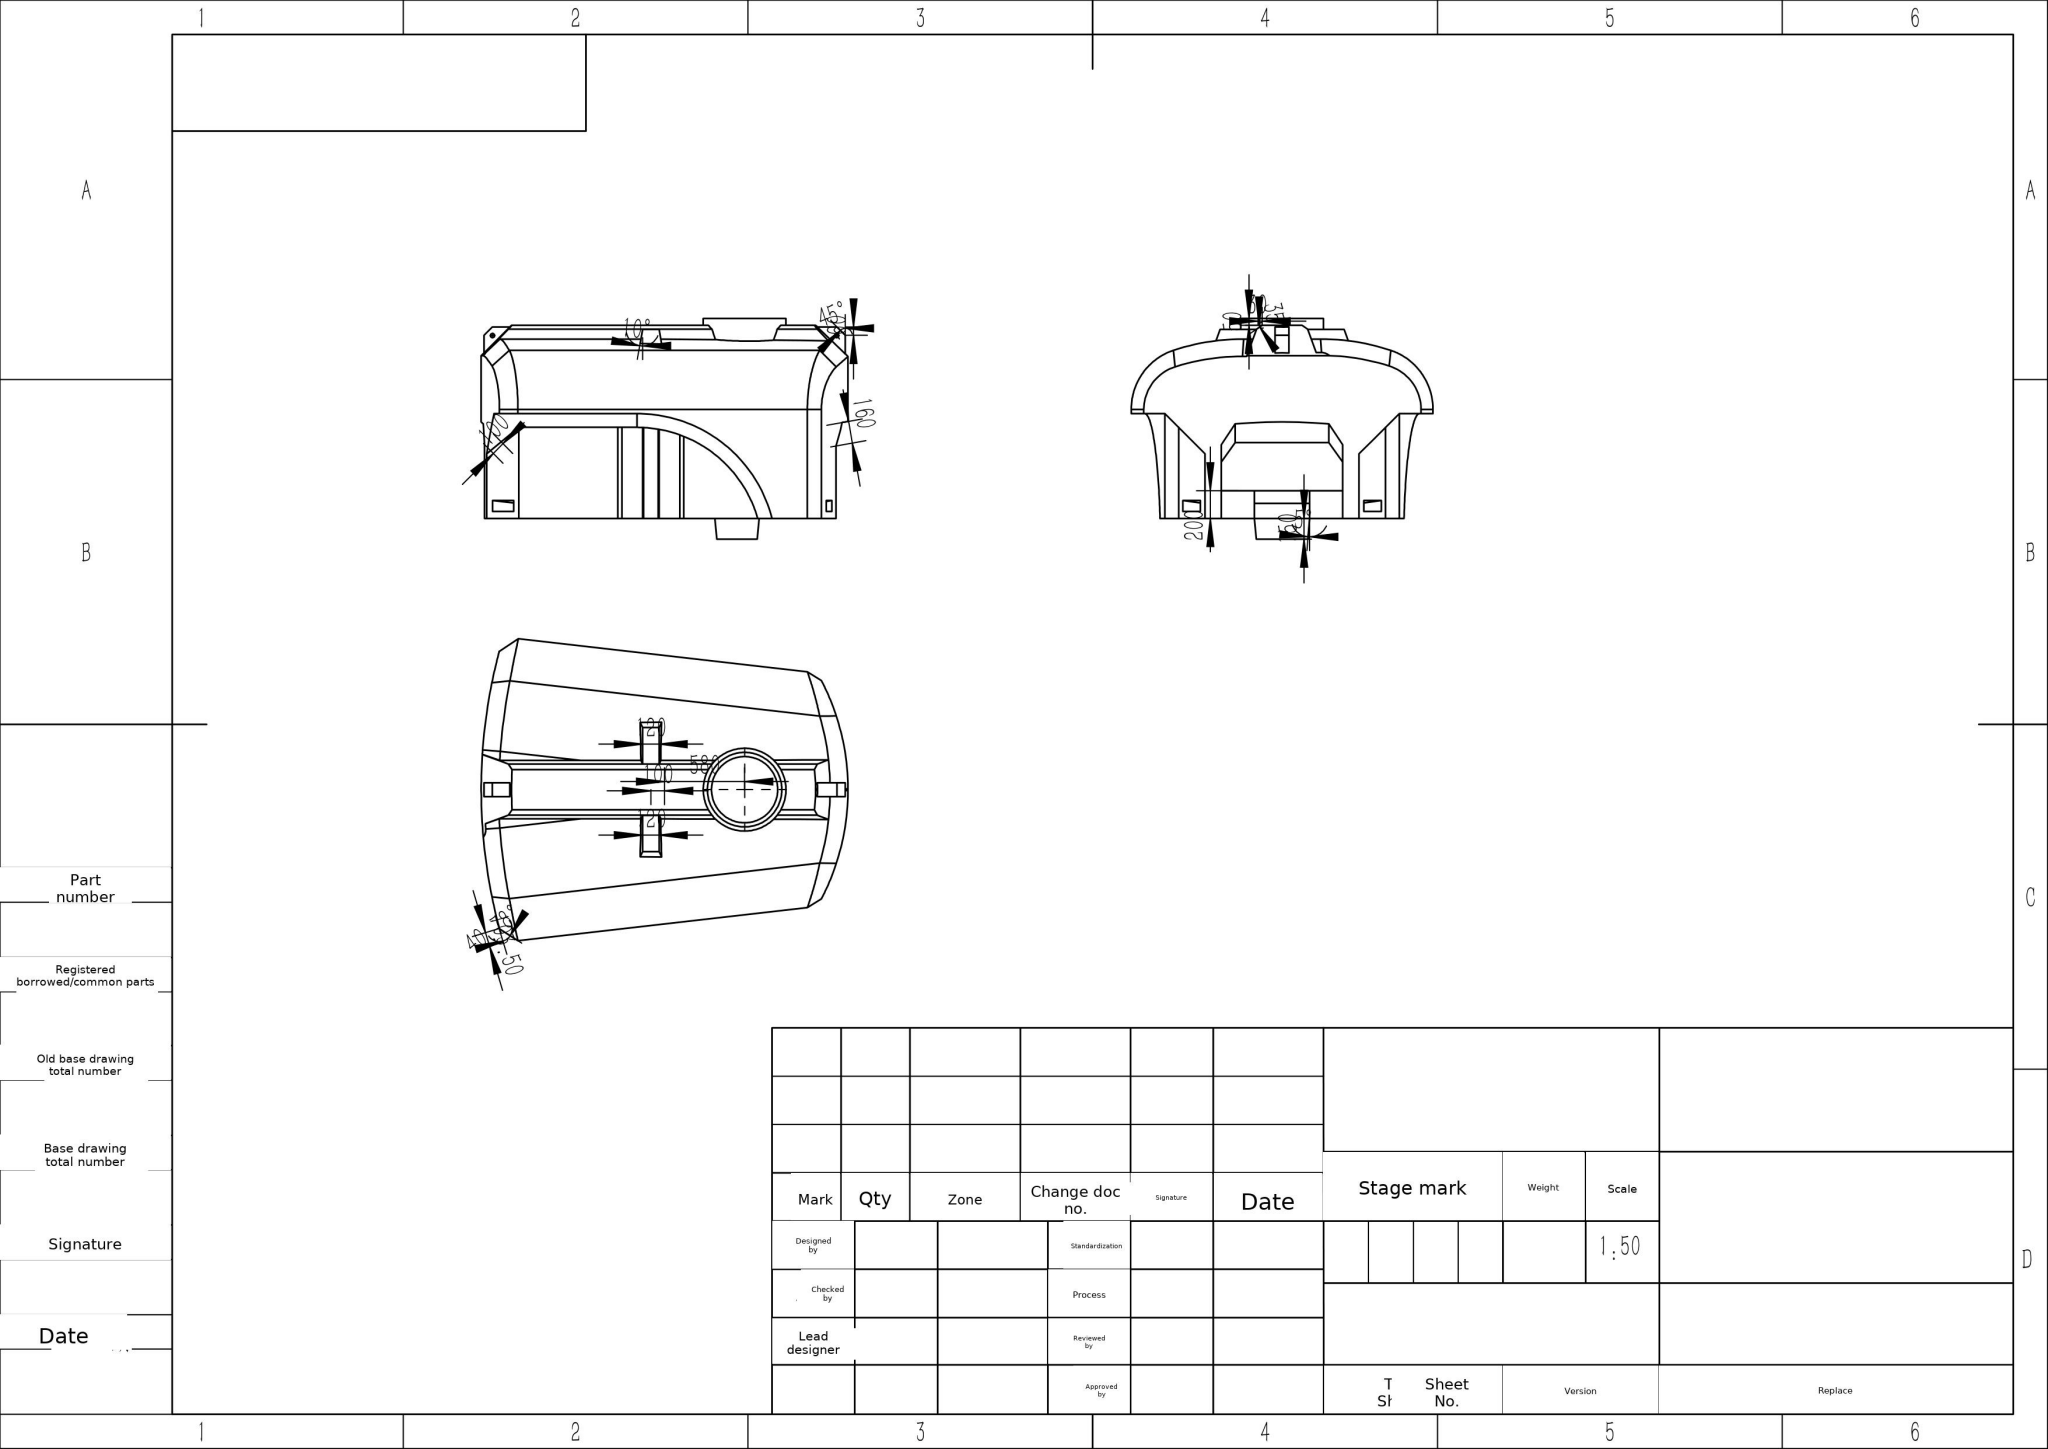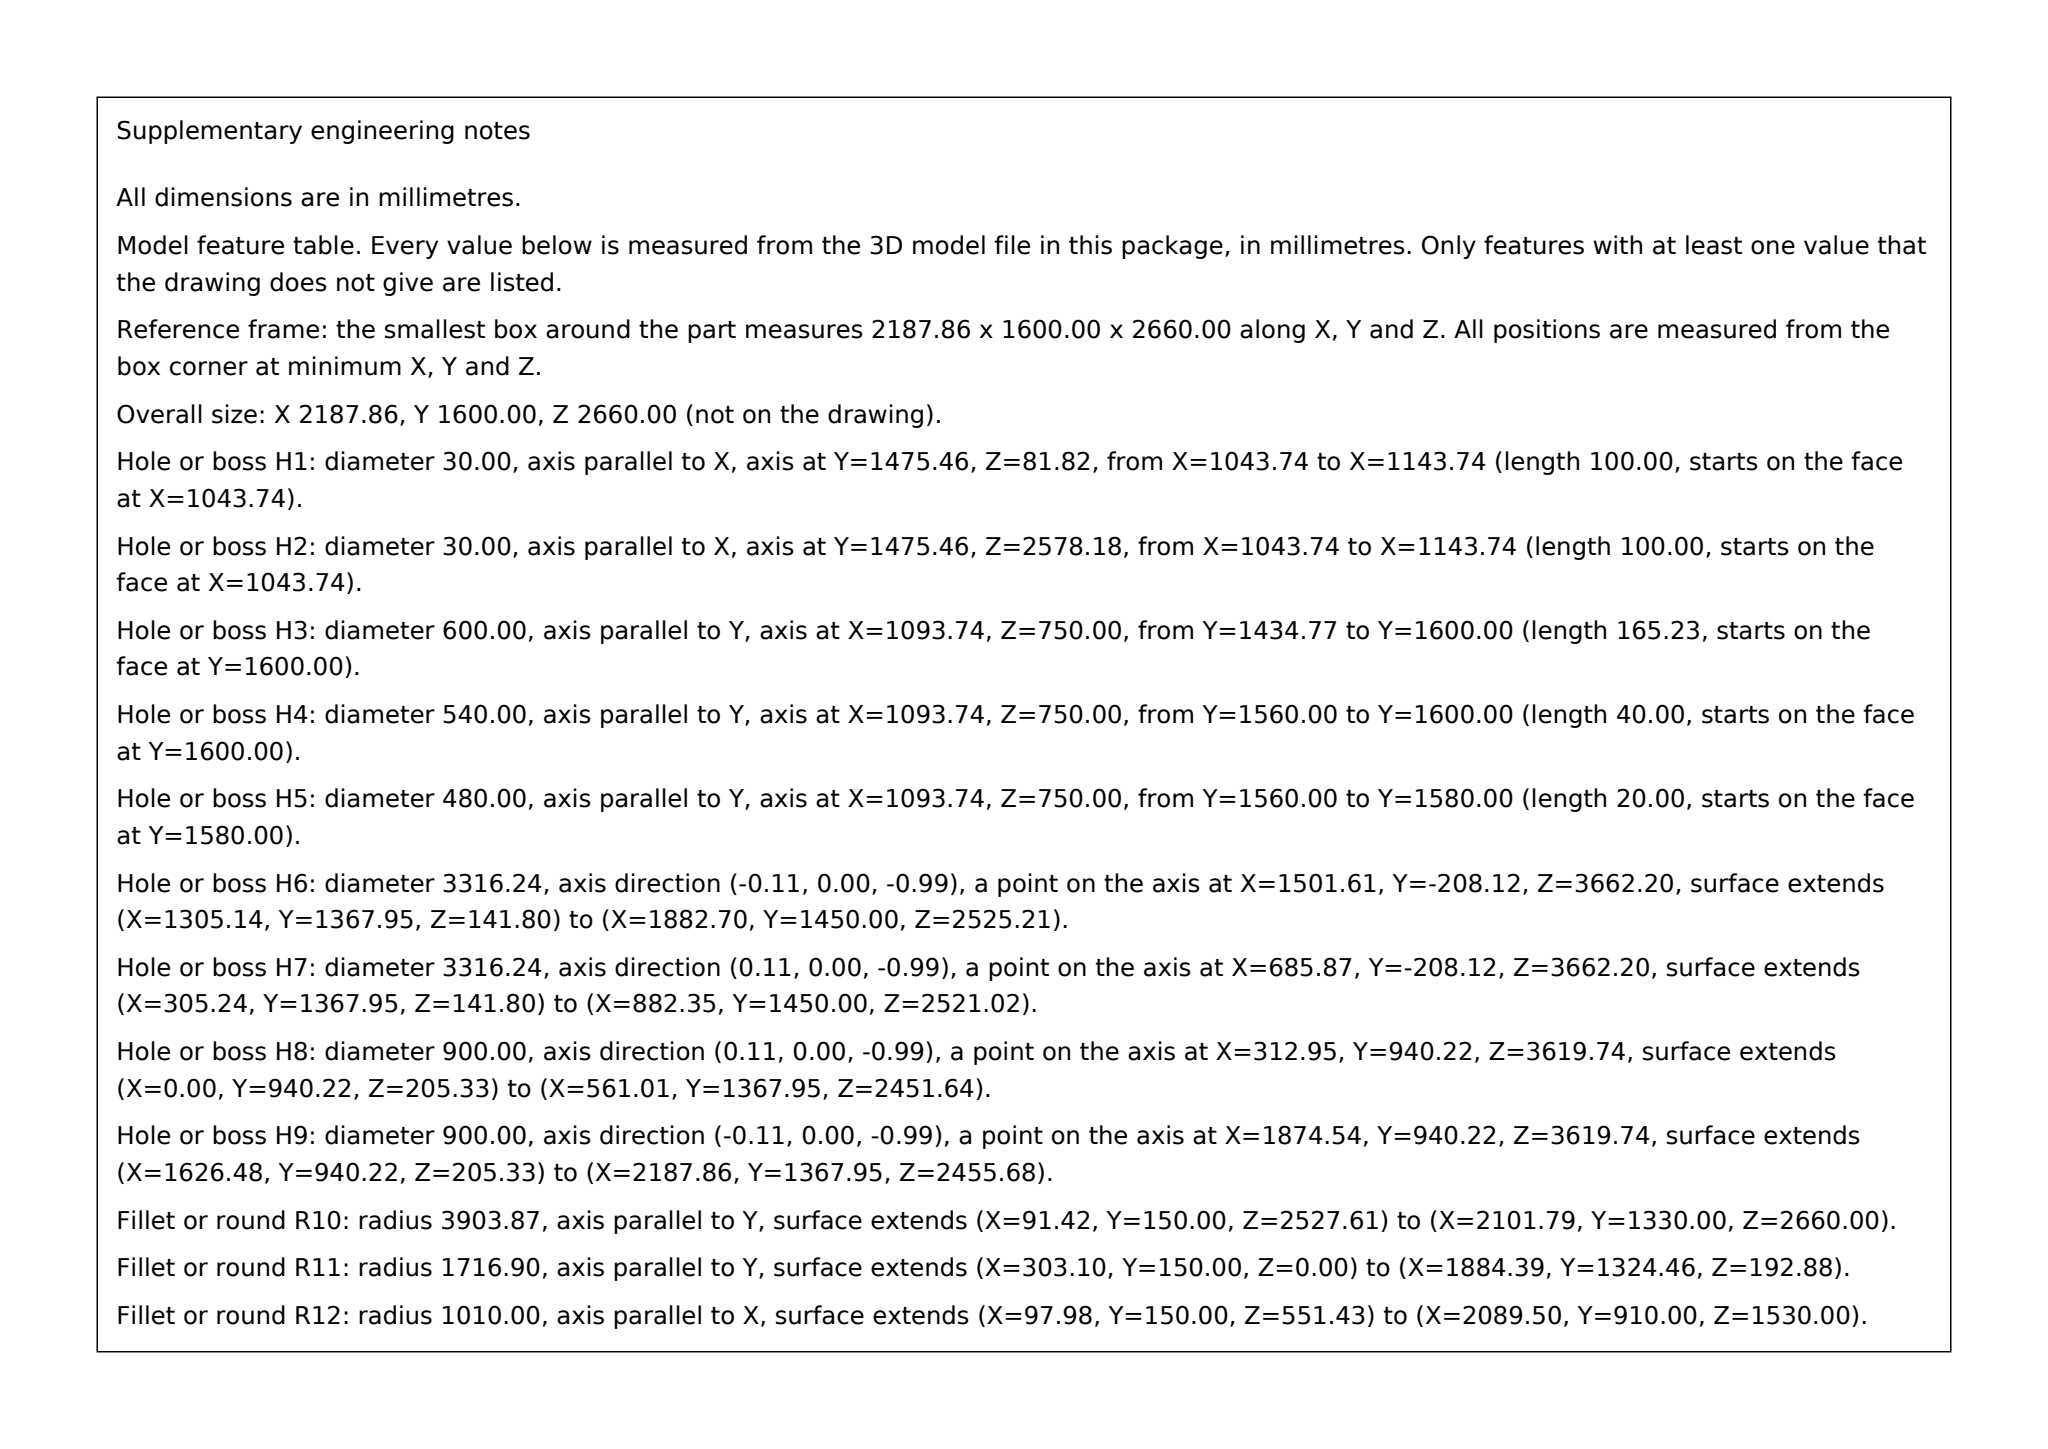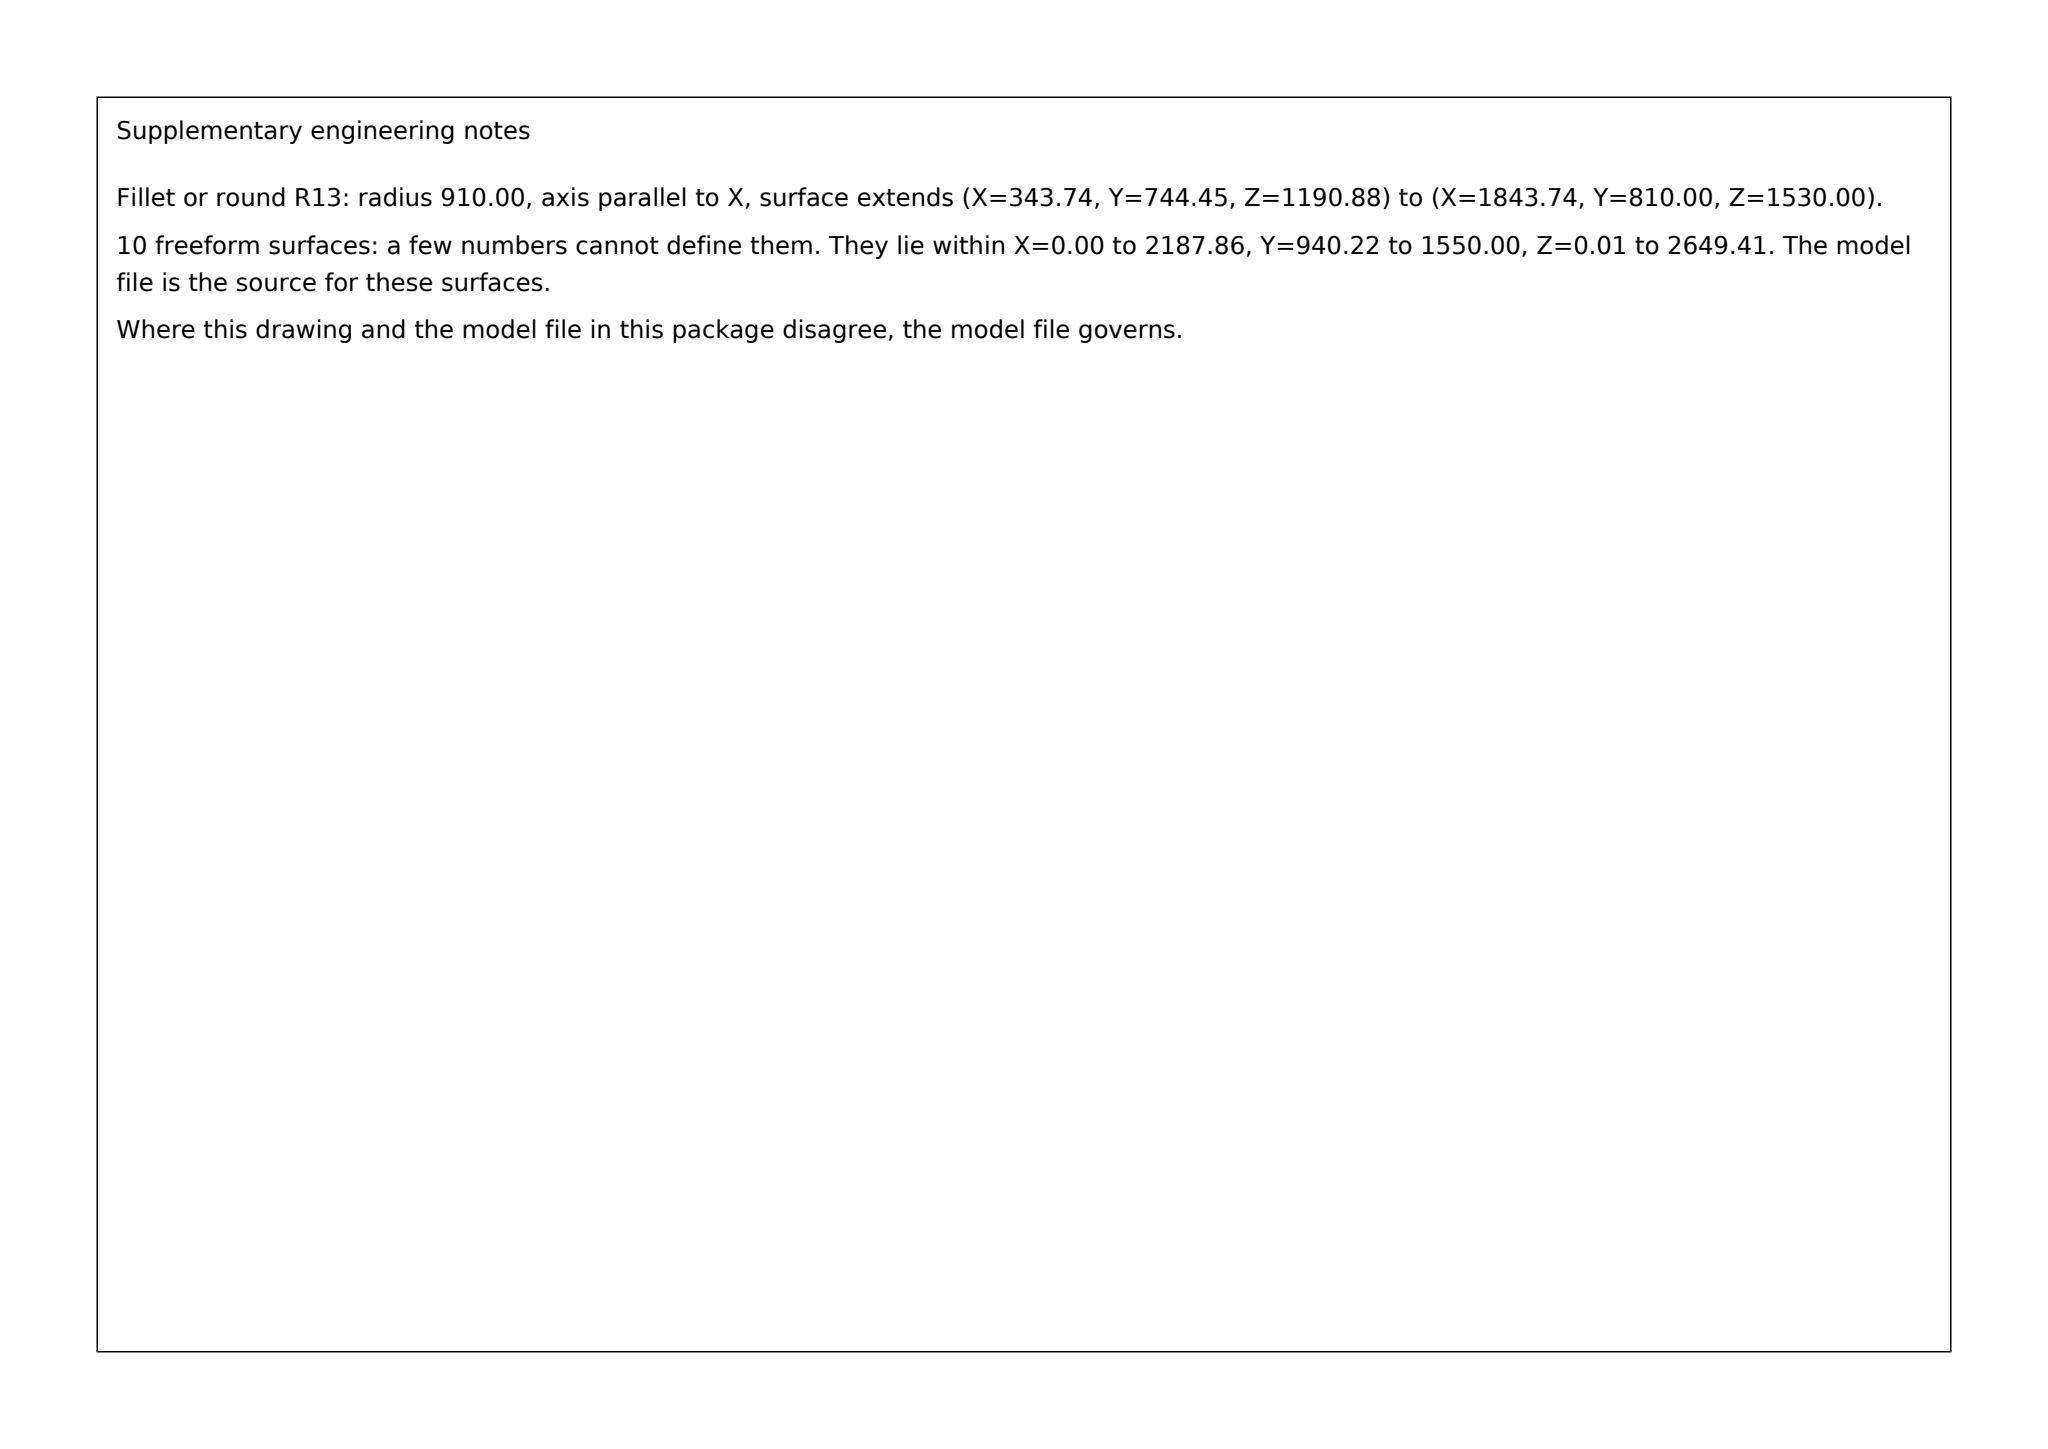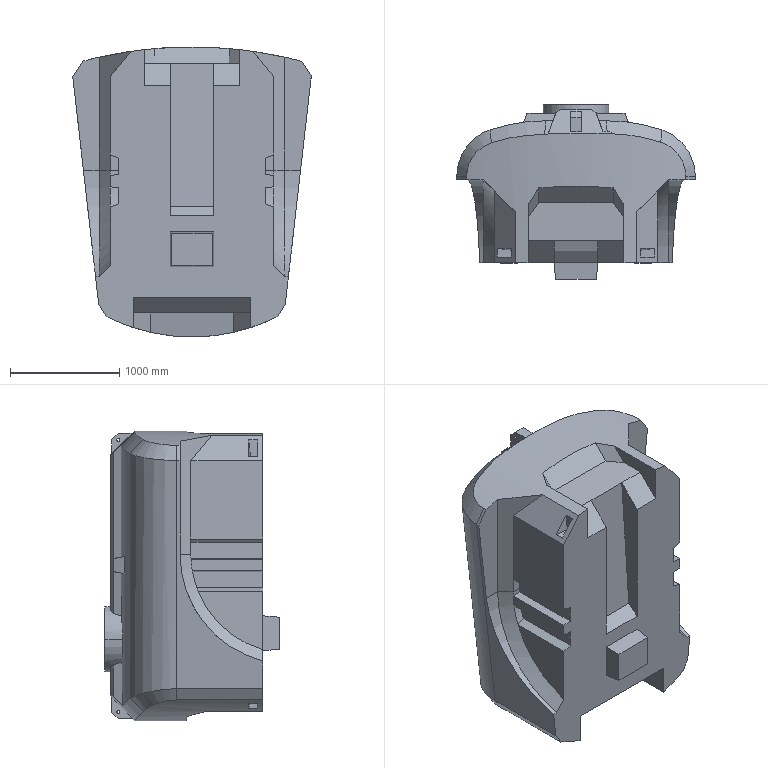Part | SolidWorks | mm | 1 solid | 147 faces | box 2187.86 x 1600 x 2660 mm | volume 5114602708 mm3 | plane 108 | cylinder 22 | spline 10 | cone 7 | commonest cylinder face diameters 30 x4 1820 x4 480 x2 540 x2 600 x2 3316.237 x2 2020 x2 900 x2